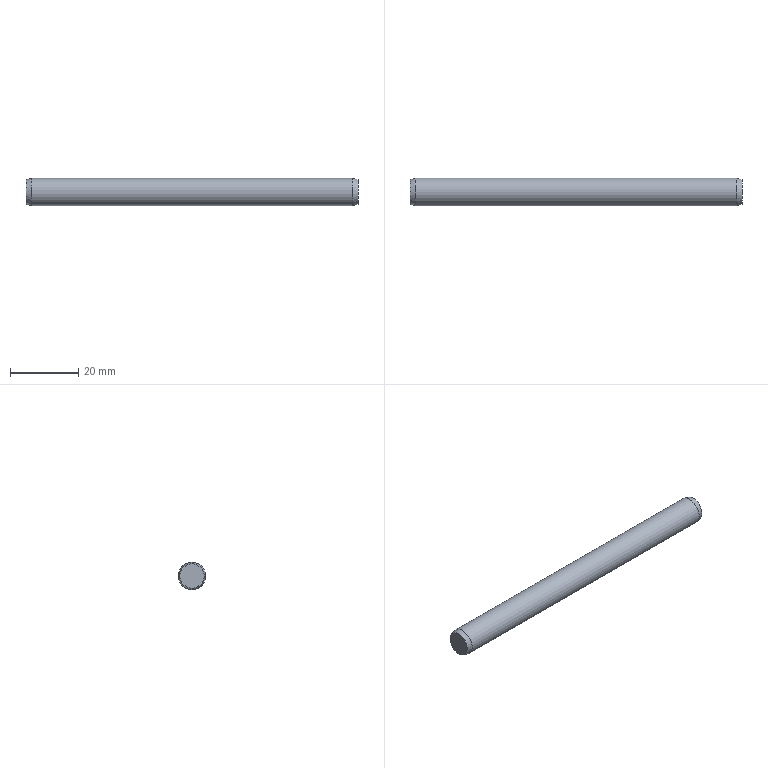Component | NX | HINGE | 1 solid | 5 faces | box 97 x 8 x 8 mm | volume 4859 mm3 | plane 2 | cone 2 | cylinder 1 | commonest cylinder face diameters 8 x1
STEP:
#1=CARTESIAN_POINT('',(0.,0.,0.));
#2=DIRECTION('',(0.,0.,1.));
#3=DIRECTION('',(1.,0.,0.));
#4=AXIS2_PLACEMENT_3D('',#1,#2,#3);
#5=CARTESIAN_POINT('',(397.101,-67.,105.571));
#6=VERTEX_POINT('',#5);
#7=CARTESIAN_POINT('',(397.101,-67.,102.));
#8=DIRECTION('',(1.,0.,0.));
#9=DIRECTION('',(0.,0.,1.));
#10=AXIS2_PLACEMENT_3D('',#7,#8,#9);
#11=CIRCLE('',#10,3.571);
#12=CARTESIAN_POINT('',(397.101,-67.,102.));
#13=DIRECTION('',(1.,0.,0.));
#14=DIRECTION('',(0.,0.,1.));
#15=AXIS2_PLACEMENT_3D('',#12,#13,#14);
#16=PLANE('',#15);
#17=CARTESIAN_POINT('',(0.,0.));
#18=DIRECTION('',(1.,0.));
#19=AXIS2_PLACEMENT_2D('',#17,#18);
#20=CIRCLE('',#19,3.571);
#21=(GEOMETRIC_REPRESENTATION_CONTEXT(2)PARAMETRIC_REPRESENTATION_CONTEXT()REPRESENTATION_CONTEXT('',''));
#22=DEFINITIONAL_REPRESENTATION('',(#20),#21);
#23=PCURVE('',#16,#22);
#24=CARTESIAN_POINT('',(397.101,-67.,102.));
#25=DIRECTION('',(-1.,0.,0.));
#26=DIRECTION('',(0.,0.,-1.));
#27=AXIS2_PLACEMENT_3D('',#24,#25,#26);
#28=CONICAL_SURFACE('',#27,3.571,0.2618);
#29=CARTESIAN_POINT('',(9.425,-0.));
#30=DIRECTION('',(-1.,0.));
#31=VECTOR('',#30,1.);
#32=LINE('',#29,#31);
#33=(GEOMETRIC_REPRESENTATION_CONTEXT(2)PARAMETRIC_REPRESENTATION_CONTEXT()REPRESENTATION_CONTEXT('',''));
#34=DEFINITIONAL_REPRESENTATION('',(#32),#33);
#35=PCURVE('',#28,#34);
#36=SURFACE_CURVE('',#11,(#23,#35),.PCURVE_S1.);
#37=EDGE_CURVE('',#6,#6,#36,.T.);
#38=ORIENTED_EDGE('',*,*,#37,.T.);
#39=EDGE_LOOP('',(#38));
#40=FACE_BOUND('',#39,.T.);
#41=ADVANCED_FACE('',(#40),#16,.T.);
#42=CARTESIAN_POINT('',(395.501,-67.,106.));
#43=VERTEX_POINT('',#42);
#44=CARTESIAN_POINT('',(395.501,-67.,102.));
#45=DIRECTION('',(1.,0.,0.));
#46=DIRECTION('',(0.,0.,1.));
#47=AXIS2_PLACEMENT_3D('',#44,#45,#46);
#48=CIRCLE('',#47,4.);
#49=CARTESIAN_POINT('',(9.425,1.6));
#50=DIRECTION('',(-1.,0.));
#51=VECTOR('',#50,1.);
#52=LINE('',#49,#51);
#53=(GEOMETRIC_REPRESENTATION_CONTEXT(2)PARAMETRIC_REPRESENTATION_CONTEXT()REPRESENTATION_CONTEXT('',''));
#54=DEFINITIONAL_REPRESENTATION('',(#52),#53);
#55=PCURVE('',#28,#54);
#56=CARTESIAN_POINT('',(300.101,-67.,102.));
#57=DIRECTION('',(1.,0.,0.));
#58=DIRECTION('',(0.,0.,1.));
#59=AXIS2_PLACEMENT_3D('',#56,#57,#58);
#60=CYLINDRICAL_SURFACE('',#59,4.);
#61=CARTESIAN_POINT('',(0.,95.4));
#62=DIRECTION('',(1.,0.));
#63=VECTOR('',#62,1.);
#64=LINE('',#61,#63);
#65=(GEOMETRIC_REPRESENTATION_CONTEXT(2)PARAMETRIC_REPRESENTATION_CONTEXT()REPRESENTATION_CONTEXT('',''));
#66=DEFINITIONAL_REPRESENTATION('',(#64),#65);
#67=PCURVE('',#60,#66);
#68=SURFACE_CURVE('',#48,(#55,#67),.PCURVE_S1.);
#69=EDGE_CURVE('',#43,#43,#68,.T.);
#70=ORIENTED_EDGE('',*,*,#69,.T.);
#71=CARTESIAN_POINT('',(397.101,-67.,105.571));
#72=CARTESIAN_POINT('',(395.501,-67.,106.));
#73=B_SPLINE_CURVE_WITH_KNOTS('',1,(#71,#72),.UNSPECIFIED.,.F.,.F.,(2,2),(-0.,1.656),.PIECEWISE_BEZIER_KNOTS.);
#74=CARTESIAN_POINT('',(3.142,0.));
#75=DIRECTION('',(0.,1.));
#76=VECTOR('',#75,1.);
#77=LINE('',#74,#76);
#78=(GEOMETRIC_REPRESENTATION_CONTEXT(2)PARAMETRIC_REPRESENTATION_CONTEXT()REPRESENTATION_CONTEXT('',''));
#79=DEFINITIONAL_REPRESENTATION('',(#77),#78);
#80=PCURVE('',#28,#79);
#81=CARTESIAN_POINT('',(9.425,0.));
#82=DIRECTION('',(0.,1.));
#83=VECTOR('',#82,1.);
#84=LINE('',#81,#83);
#85=(GEOMETRIC_REPRESENTATION_CONTEXT(2)PARAMETRIC_REPRESENTATION_CONTEXT()REPRESENTATION_CONTEXT('',''));
#86=DEFINITIONAL_REPRESENTATION('',(#84),#85);
#87=PCURVE('',#28,#86);
#88=SEAM_CURVE('',#73,(#80,#87),.PCURVE_S1.);
#89=EDGE_CURVE('',#6,#43,#88,.T.);
#90=ORIENTED_EDGE('',*,*,#89,.F.);
#91=ORIENTED_EDGE('',*,*,#37,.F.);
#92=ORIENTED_EDGE('',*,*,#89,.T.);
#93=EDGE_LOOP('',(#70,#90,#91,#92));
#94=FACE_BOUND('',#93,.T.);
#95=ADVANCED_FACE('',(#94),#28,.T.);
#96=CARTESIAN_POINT('',(301.701,-67.,106.));
#97=VERTEX_POINT('',#96);
#98=CARTESIAN_POINT('',(301.701,-67.,102.));
#99=DIRECTION('',(1.,0.,0.));
#100=DIRECTION('',(0.,0.,1.));
#101=AXIS2_PLACEMENT_3D('',#98,#99,#100);
#102=CIRCLE('',#101,4.);
#103=CARTESIAN_POINT('',(0.,1.6));
#104=DIRECTION('',(1.,0.));
#105=VECTOR('',#104,1.);
#106=LINE('',#103,#105);
#107=(GEOMETRIC_REPRESENTATION_CONTEXT(2)PARAMETRIC_REPRESENTATION_CONTEXT()REPRESENTATION_CONTEXT('',''));
#108=DEFINITIONAL_REPRESENTATION('',(#106),#107);
#109=PCURVE('',#60,#108);
#110=CARTESIAN_POINT('',(301.701,-67.,102.));
#111=DIRECTION('',(1.,0.,0.));
#112=DIRECTION('',(0.,0.,1.));
#113=AXIS2_PLACEMENT_3D('',#110,#111,#112);
#114=CONICAL_SURFACE('',#113,4.,0.2618);
#115=CARTESIAN_POINT('',(0.,-0.));
#116=DIRECTION('',(1.,0.));
#117=VECTOR('',#116,1.);
#118=LINE('',#115,#117);
#119=(GEOMETRIC_REPRESENTATION_CONTEXT(2)PARAMETRIC_REPRESENTATION_CONTEXT()REPRESENTATION_CONTEXT('',''));
#120=DEFINITIONAL_REPRESENTATION('',(#118),#119);
#121=PCURVE('',#114,#120);
#122=SURFACE_CURVE('',#102,(#109,#121),.PCURVE_S1.);
#123=EDGE_CURVE('',#97,#97,#122,.T.);
#124=ORIENTED_EDGE('',*,*,#123,.T.);
#125=CARTESIAN_POINT('',(301.701,-67.,106.));
#126=CARTESIAN_POINT('',(395.501,-67.,106.));
#127=B_SPLINE_CURVE_WITH_KNOTS('',1,(#125,#126),.UNSPECIFIED.,.F.,.F.,(2,2),(1.6,95.4),.PIECEWISE_BEZIER_KNOTS.);
#128=CARTESIAN_POINT('',(6.283,0.));
#129=DIRECTION('',(0.,1.));
#130=VECTOR('',#129,1.);
#131=LINE('',#128,#130);
#132=(GEOMETRIC_REPRESENTATION_CONTEXT(2)PARAMETRIC_REPRESENTATION_CONTEXT()REPRESENTATION_CONTEXT('',''));
#133=DEFINITIONAL_REPRESENTATION('',(#131),#132);
#134=PCURVE('',#60,#133);
#135=CARTESIAN_POINT('',(0.,0.));
#136=DIRECTION('',(0.,1.));
#137=VECTOR('',#136,1.);
#138=LINE('',#135,#137);
#139=(GEOMETRIC_REPRESENTATION_CONTEXT(2)PARAMETRIC_REPRESENTATION_CONTEXT()REPRESENTATION_CONTEXT('',''));
#140=DEFINITIONAL_REPRESENTATION('',(#138),#139);
#141=PCURVE('',#60,#140);
#142=SEAM_CURVE('',#127,(#134,#141),.PCURVE_S1.);
#143=EDGE_CURVE('',#97,#43,#142,.T.);
#144=ORIENTED_EDGE('',*,*,#143,.T.);
#145=ORIENTED_EDGE('',*,*,#69,.F.);
#146=ORIENTED_EDGE('',*,*,#143,.F.);
#147=EDGE_LOOP('',(#124,#144,#145,#146));
#148=FACE_BOUND('',#147,.T.);
#149=ADVANCED_FACE('',(#148),#60,.T.);
#150=CARTESIAN_POINT('',(300.101,-67.,105.571));
#151=VERTEX_POINT('',#150);
#152=CARTESIAN_POINT('',(300.101,-67.,102.));
#153=DIRECTION('',(1.,0.,0.));
#154=DIRECTION('',(0.,0.,1.));
#155=AXIS2_PLACEMENT_3D('',#152,#153,#154);
#156=CIRCLE('',#155,3.571);
#157=CARTESIAN_POINT('',(0.,-1.6));
#158=DIRECTION('',(1.,0.));
#159=VECTOR('',#158,1.);
#160=LINE('',#157,#159);
#161=(GEOMETRIC_REPRESENTATION_CONTEXT(2)PARAMETRIC_REPRESENTATION_CONTEXT()REPRESENTATION_CONTEXT('',''));
#162=DEFINITIONAL_REPRESENTATION('',(#160),#161);
#163=PCURVE('',#114,#162);
#164=CARTESIAN_POINT('',(300.101,-67.,98.429));
#165=DIRECTION('',(-1.,0.,0.));
#166=DIRECTION('',(0.,0.,-1.));
#167=AXIS2_PLACEMENT_3D('',#164,#165,#166);
#168=PLANE('',#167);
#169=CARTESIAN_POINT('',(-7.143,0.));
#170=CARTESIAN_POINT('',(-7.143,6.186));
#171=CARTESIAN_POINT('',(-1.786,3.093));
#172=CARTESIAN_POINT('',(3.571,0.));
#173=CARTESIAN_POINT('',(-1.786,-3.093));
#174=CARTESIAN_POINT('',(-7.143,-6.186));
#175=CARTESIAN_POINT('',(-7.143,0.));
#176=(BOUNDED_CURVE()B_SPLINE_CURVE(2,(#169,#170,#171,#172,#173,#174,#175),.UNSPECIFIED.,.T.,.F.)B_SPLINE_CURVE_WITH_KNOTS((1,2,2,2,2,1),(-2.094,0.,2.094,4.189,6.283,8.378),.UNSPECIFIED.)CURVE()GEOMETRIC_REPRESENTATION_ITEM()RATIONAL_B_SPLINE_CURVE((1.,0.5,1.,0.5,1.,0.5,1.))REPRESENTATION_ITEM(''));
#177=(GEOMETRIC_REPRESENTATION_CONTEXT(2)PARAMETRIC_REPRESENTATION_CONTEXT()REPRESENTATION_CONTEXT('',''));
#178=DEFINITIONAL_REPRESENTATION('',(#176),#177);
#179=PCURVE('',#168,#178);
#180=SURFACE_CURVE('',#156,(#163,#179),.PCURVE_S1.);
#181=EDGE_CURVE('',#151,#151,#180,.T.);
#182=ORIENTED_EDGE('',*,*,#181,.T.);
#183=CARTESIAN_POINT('',(300.101,-67.,105.571));
#184=CARTESIAN_POINT('',(301.701,-67.,106.));
#185=B_SPLINE_CURVE_WITH_KNOTS('',1,(#183,#184),.UNSPECIFIED.,.F.,.F.,(2,2),(-1.656,-0.),.PIECEWISE_BEZIER_KNOTS.);
#186=CARTESIAN_POINT('',(6.283,0.));
#187=DIRECTION('',(0.,1.));
#188=VECTOR('',#187,1.);
#189=LINE('',#186,#188);
#190=(GEOMETRIC_REPRESENTATION_CONTEXT(2)PARAMETRIC_REPRESENTATION_CONTEXT()REPRESENTATION_CONTEXT('',''));
#191=DEFINITIONAL_REPRESENTATION('',(#189),#190);
#192=PCURVE('',#114,#191);
#193=CARTESIAN_POINT('',(0.,0.));
#194=DIRECTION('',(0.,1.));
#195=VECTOR('',#194,1.);
#196=LINE('',#193,#195);
#197=(GEOMETRIC_REPRESENTATION_CONTEXT(2)PARAMETRIC_REPRESENTATION_CONTEXT()REPRESENTATION_CONTEXT('',''));
#198=DEFINITIONAL_REPRESENTATION('',(#196),#197);
#199=PCURVE('',#114,#198);
#200=SEAM_CURVE('',#185,(#192,#199),.PCURVE_S1.);
#201=EDGE_CURVE('',#151,#97,#200,.T.);
#202=ORIENTED_EDGE('',*,*,#201,.T.);
#203=ORIENTED_EDGE('',*,*,#123,.F.);
#204=ORIENTED_EDGE('',*,*,#201,.F.);
#205=EDGE_LOOP('',(#182,#202,#203,#204));
#206=FACE_BOUND('',#205,.T.);
#207=ADVANCED_FACE('',(#206),#114,.T.);
#208=ORIENTED_EDGE('',*,*,#181,.F.);
#209=EDGE_LOOP('',(#208));
#210=FACE_BOUND('',#209,.T.);
#211=ADVANCED_FACE('',(#210),#168,.T.);
#212=CLOSED_SHELL('',(#41,#95,#149,#207,#211));
#213=MANIFOLD_SOLID_BREP('',#212);
#214=(LENGTH_UNIT()NAMED_UNIT(*)SI_UNIT(.MILLI.,.METRE.));
#215=UNCERTAINTY_MEASURE_WITH_UNIT(LENGTH_MEASURE(0.00001),#214,'','');
#216=(NAMED_UNIT(*)PLANE_ANGLE_UNIT()SI_UNIT($,.RADIAN.));
#217=(NAMED_UNIT(*)SI_UNIT($,.STERADIAN.)SOLID_ANGLE_UNIT());
#218=(GEOMETRIC_REPRESENTATION_CONTEXT(3)GLOBAL_UNCERTAINTY_ASSIGNED_CONTEXT((#215))GLOBAL_UNIT_ASSIGNED_CONTEXT((#214,#216,#217))REPRESENTATION_CONTEXT('',''));
#219=ADVANCED_BREP_SHAPE_REPRESENTATION('',(#4,#213),#218);